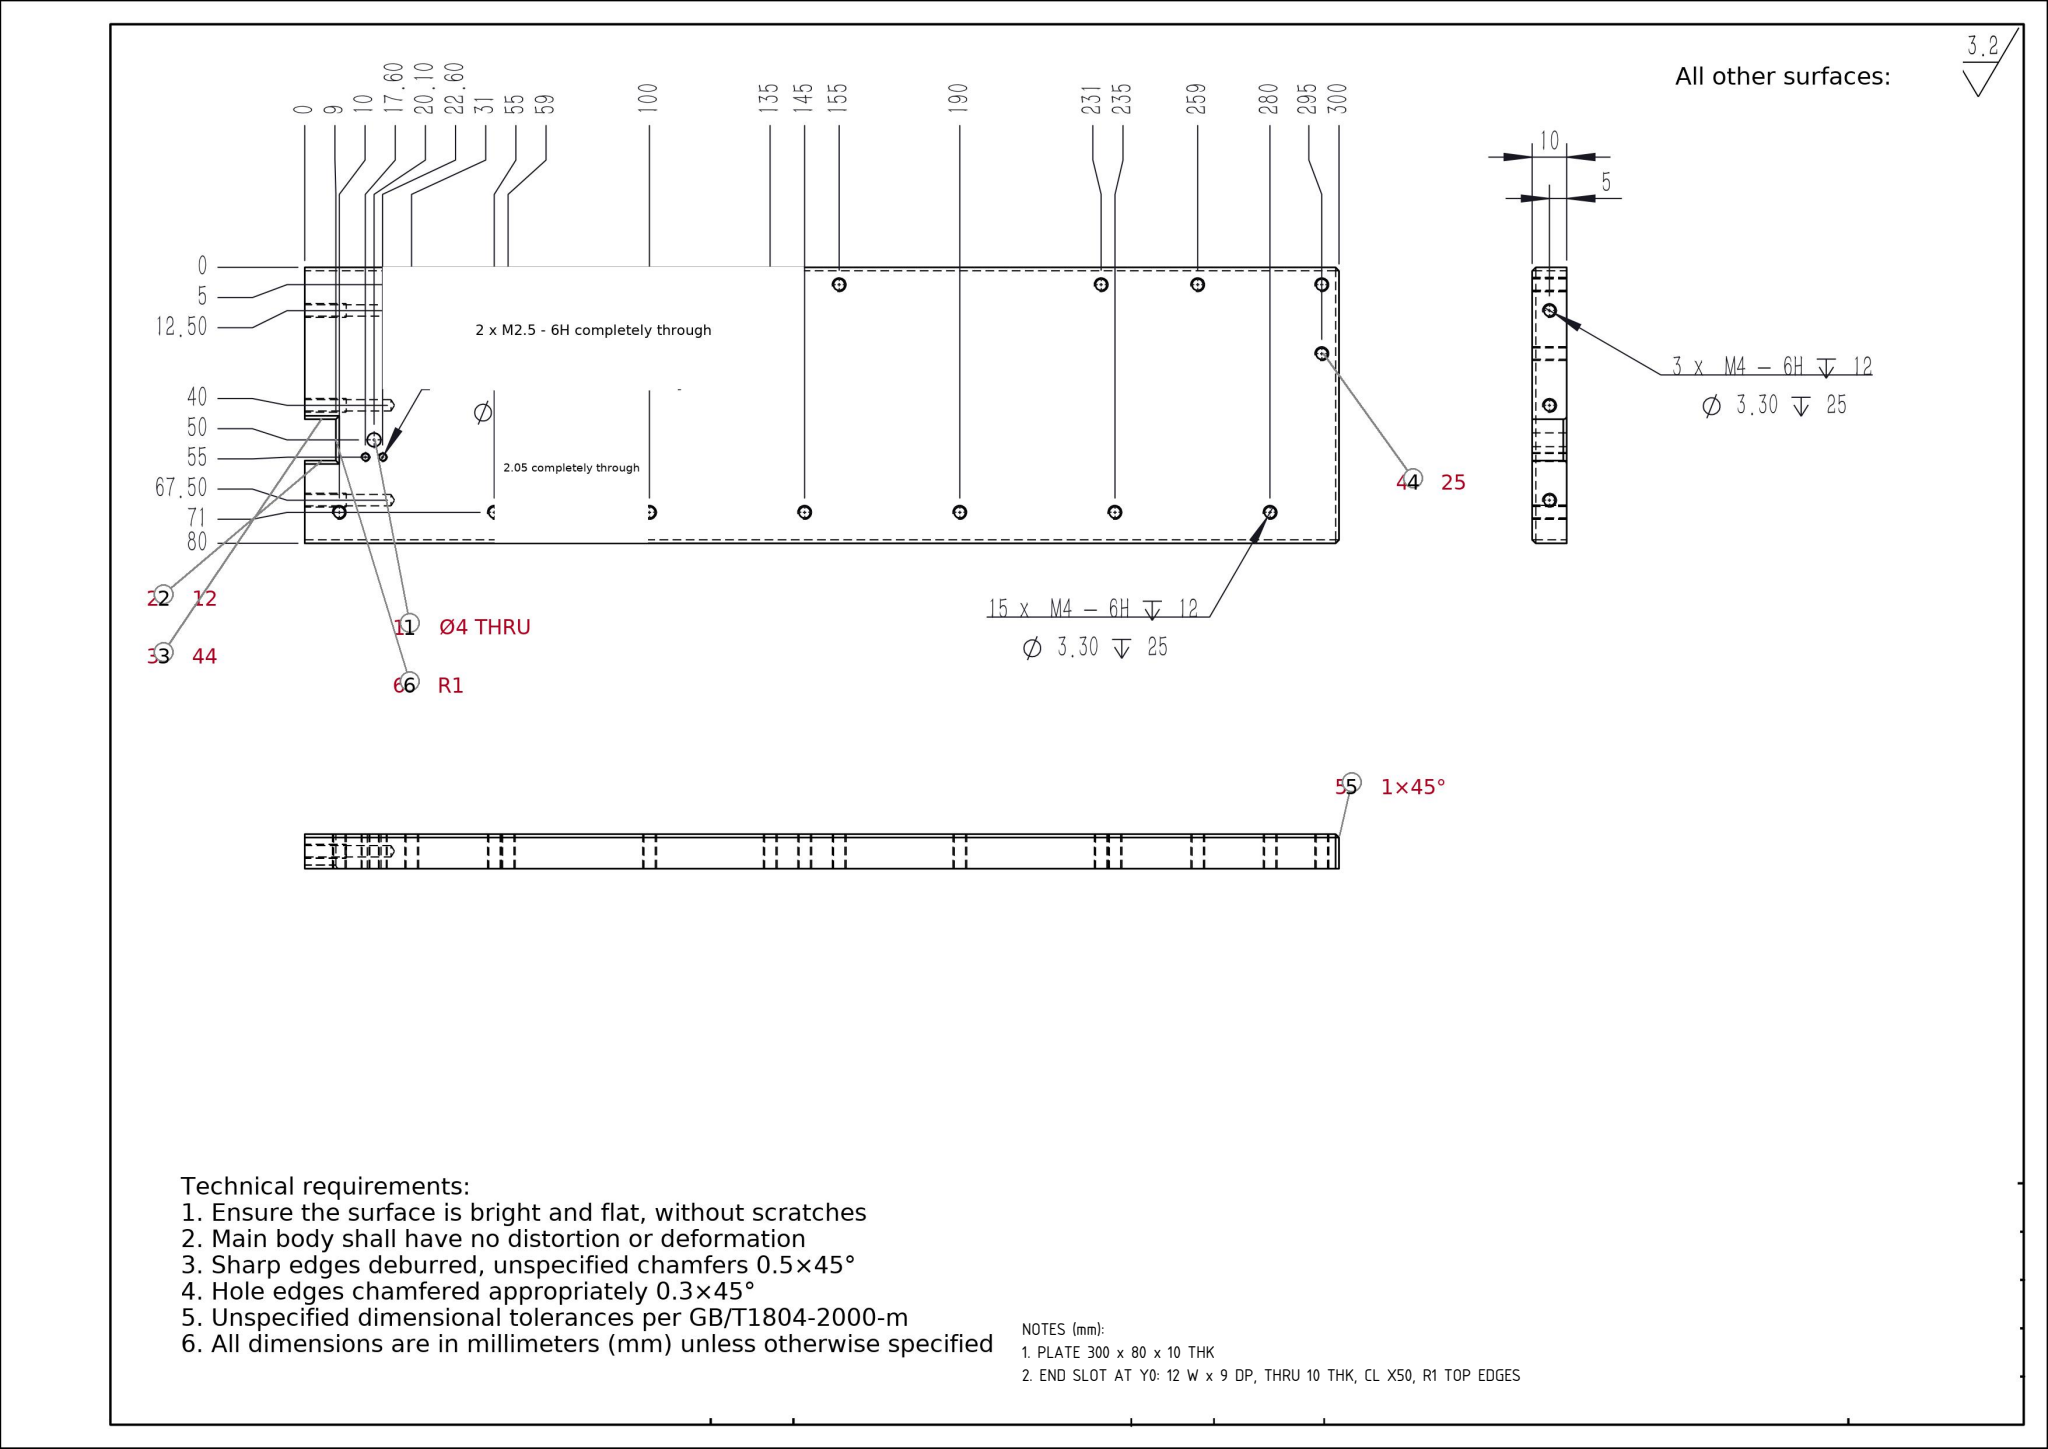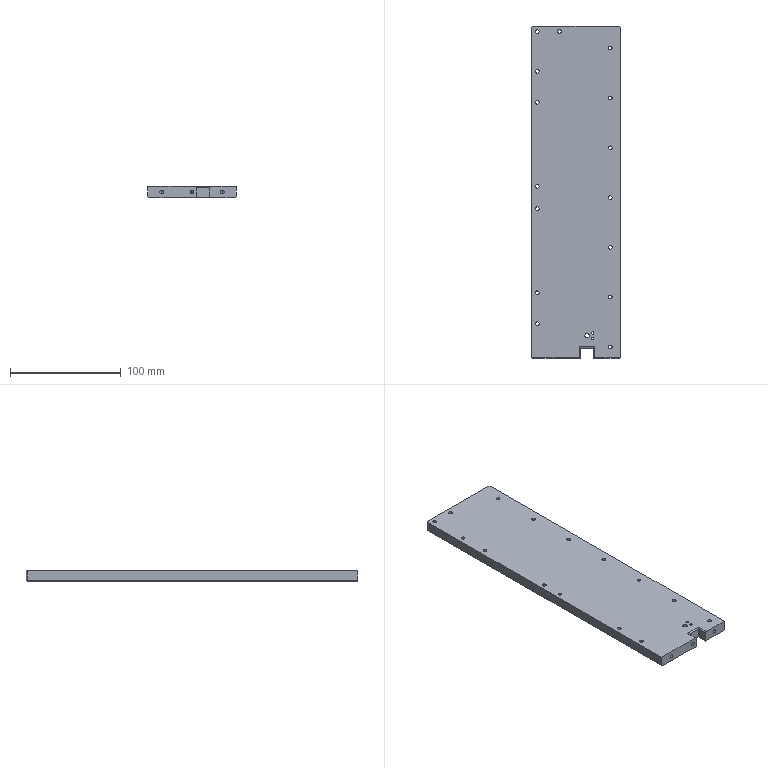Part | SolidWorks | mm | 1 solid | 68 faces | box 80 x 300 x 10 mm | volume 236440 mm3 | cylinder 45 | plane 17 | cone 6 | commonest cylinder face diameters 3.3 x36 2.05 x4 2 x3 4 x2
Drawing notes:
PLATE 300 x 80 x 10 THK | from the solid: bbox_xyz 80 x 300 x 10
END SLOT AT Y0: 12 W x 9 DP, THRU 10 THK, CL X50, R1 TOP EDGES | from the solid: Planes x=44 & x=56 (12 wide), y=9 slot bottom, y=0 end face split; z=0/z=10 only = thru 10 thk; slot mid x=50 matches Ø4 THRU at x=50, y=20.1; Ø2 cyls at x=43/57 and y=10, z=9 = R1 edges
build123d program:
from build123d import *

# Parameters (mm, degrees)
SKETCH1_W             = 80
SKETCH1_H             = 300
BOSS_EXTRUDE1_DEPTH   = 10
M4_TAPPED_HOLE1_D     = 3.3
M4_TAPPED_HOLE1_DEPTH = 25
M4_TAPPED_HOLE1_TIP   = 0.9914
M4_TAPPED_HOLE2_D     = 3.3
M4_TAPPED_HOLE2_DEPTH = 25
M4_TAPPED_HOLE2_TIP   = 0.9914
CHAMFER1_SIZE         = 1
SKETCH6_W             = 12
SKETCH6_H             = 9
CUT_EXTRUDE1_DEPTH    = 10
FILLET1_R             = 1
SKETCH7_R             = 2
CUT_EXTRUDE2_DEPTH    = 20
M2_5_TAPPED_HOLE1_D   = 2.05


with BuildPart() as part:
    # Sketch1 → Boss-Extrude1 (new body)
    with BuildSketch(Plane.XY):
        Rectangle(SKETCH1_W, SKETCH1_H)
    extrude(amount=BOSS_EXTRUDE1_DEPTH)

    # M4 Tapped Hole1
    with Locations(Plane.XY.offset(10)):
        with Locations((-15, 145), (-35, 145), (-35, 109), (-35, 81), (-35, 5), (-35, -15), (-35, -91), (-35, -119), (31, -140), (31, -95), (31, -50), (31, -5), (31, 40), (31, 85), (31, 130)):
            Hole(M4_TAPPED_HOLE1_D / 2, depth=M4_TAPPED_HOLE1_DEPTH)
            with Locations((0, 0, -(M4_TAPPED_HOLE1_DEPTH + M4_TAPPED_HOLE1_TIP / 2))):  # 118° drill point
                Cone(0, M4_TAPPED_HOLE1_D / 2, M4_TAPPED_HOLE1_TIP, mode=Mode.SUBTRACT)

    # M4 Tapped Hole2
    with Locations(Plane(origin=(0, -150, 0), x_dir=(-1, 0, 0), z_dir=(0, -1, 0))):
        with Locations((27.5, -5), (0, -5), (-27.5, -5)):
            Hole(M4_TAPPED_HOLE2_D / 2, depth=M4_TAPPED_HOLE2_DEPTH)
            with Locations((0, 0, -(M4_TAPPED_HOLE2_DEPTH + M4_TAPPED_HOLE2_TIP / 2))):  # 118° drill point
                Cone(0, M4_TAPPED_HOLE2_D / 2, M4_TAPPED_HOLE2_TIP, mode=Mode.SUBTRACT)

    # Chamfer1
    chamfer1_edges = [part.edges().sort_by_distance(p)[0] for p in [
        (-40, 0, 0),
        (0, 150, 0),
        (40, 0, 0),
        (-40, 150, 5),
        (40, 150, 5),
    ]]
    chamfer(chamfer1_edges, length=CHAMFER1_SIZE)

    # Sketch6 → Cut-Extrude1 (cut)
    with BuildSketch(Plane.XY.offset(10)):
        with Locations((10, -145.5)):
            Rectangle(SKETCH6_W, SKETCH6_H)
    extrude(amount=-CUT_EXTRUDE1_DEPTH, mode=Mode.SUBTRACT)

    # Fillet1
    fillet1_edges = [part.edges().sort_by_distance(p)[0] for p in [
        (4, -145.5, 10),
        (16, -145.5, 10),
        (10, -141, 10),
    ]]
    fillet(fillet1_edges, radius=FILLET1_R)

    # Sketch7 → Cut-Extrude2 (cut)
    with BuildSketch(Plane.XY.offset(10)):
        with Locations((10, -129.9)):
            Circle(SKETCH7_R)
    extrude(amount=-CUT_EXTRUDE2_DEPTH, mode=Mode.SUBTRACT)

    # M2.5 Tapped Hole1 (through all)
    with Locations(Plane.XY.offset(10)):
        with Locations((15, -127.4), (15, -132.4)):
            Hole(M2_5_TAPPED_HOLE1_D / 2)


solid = part.part